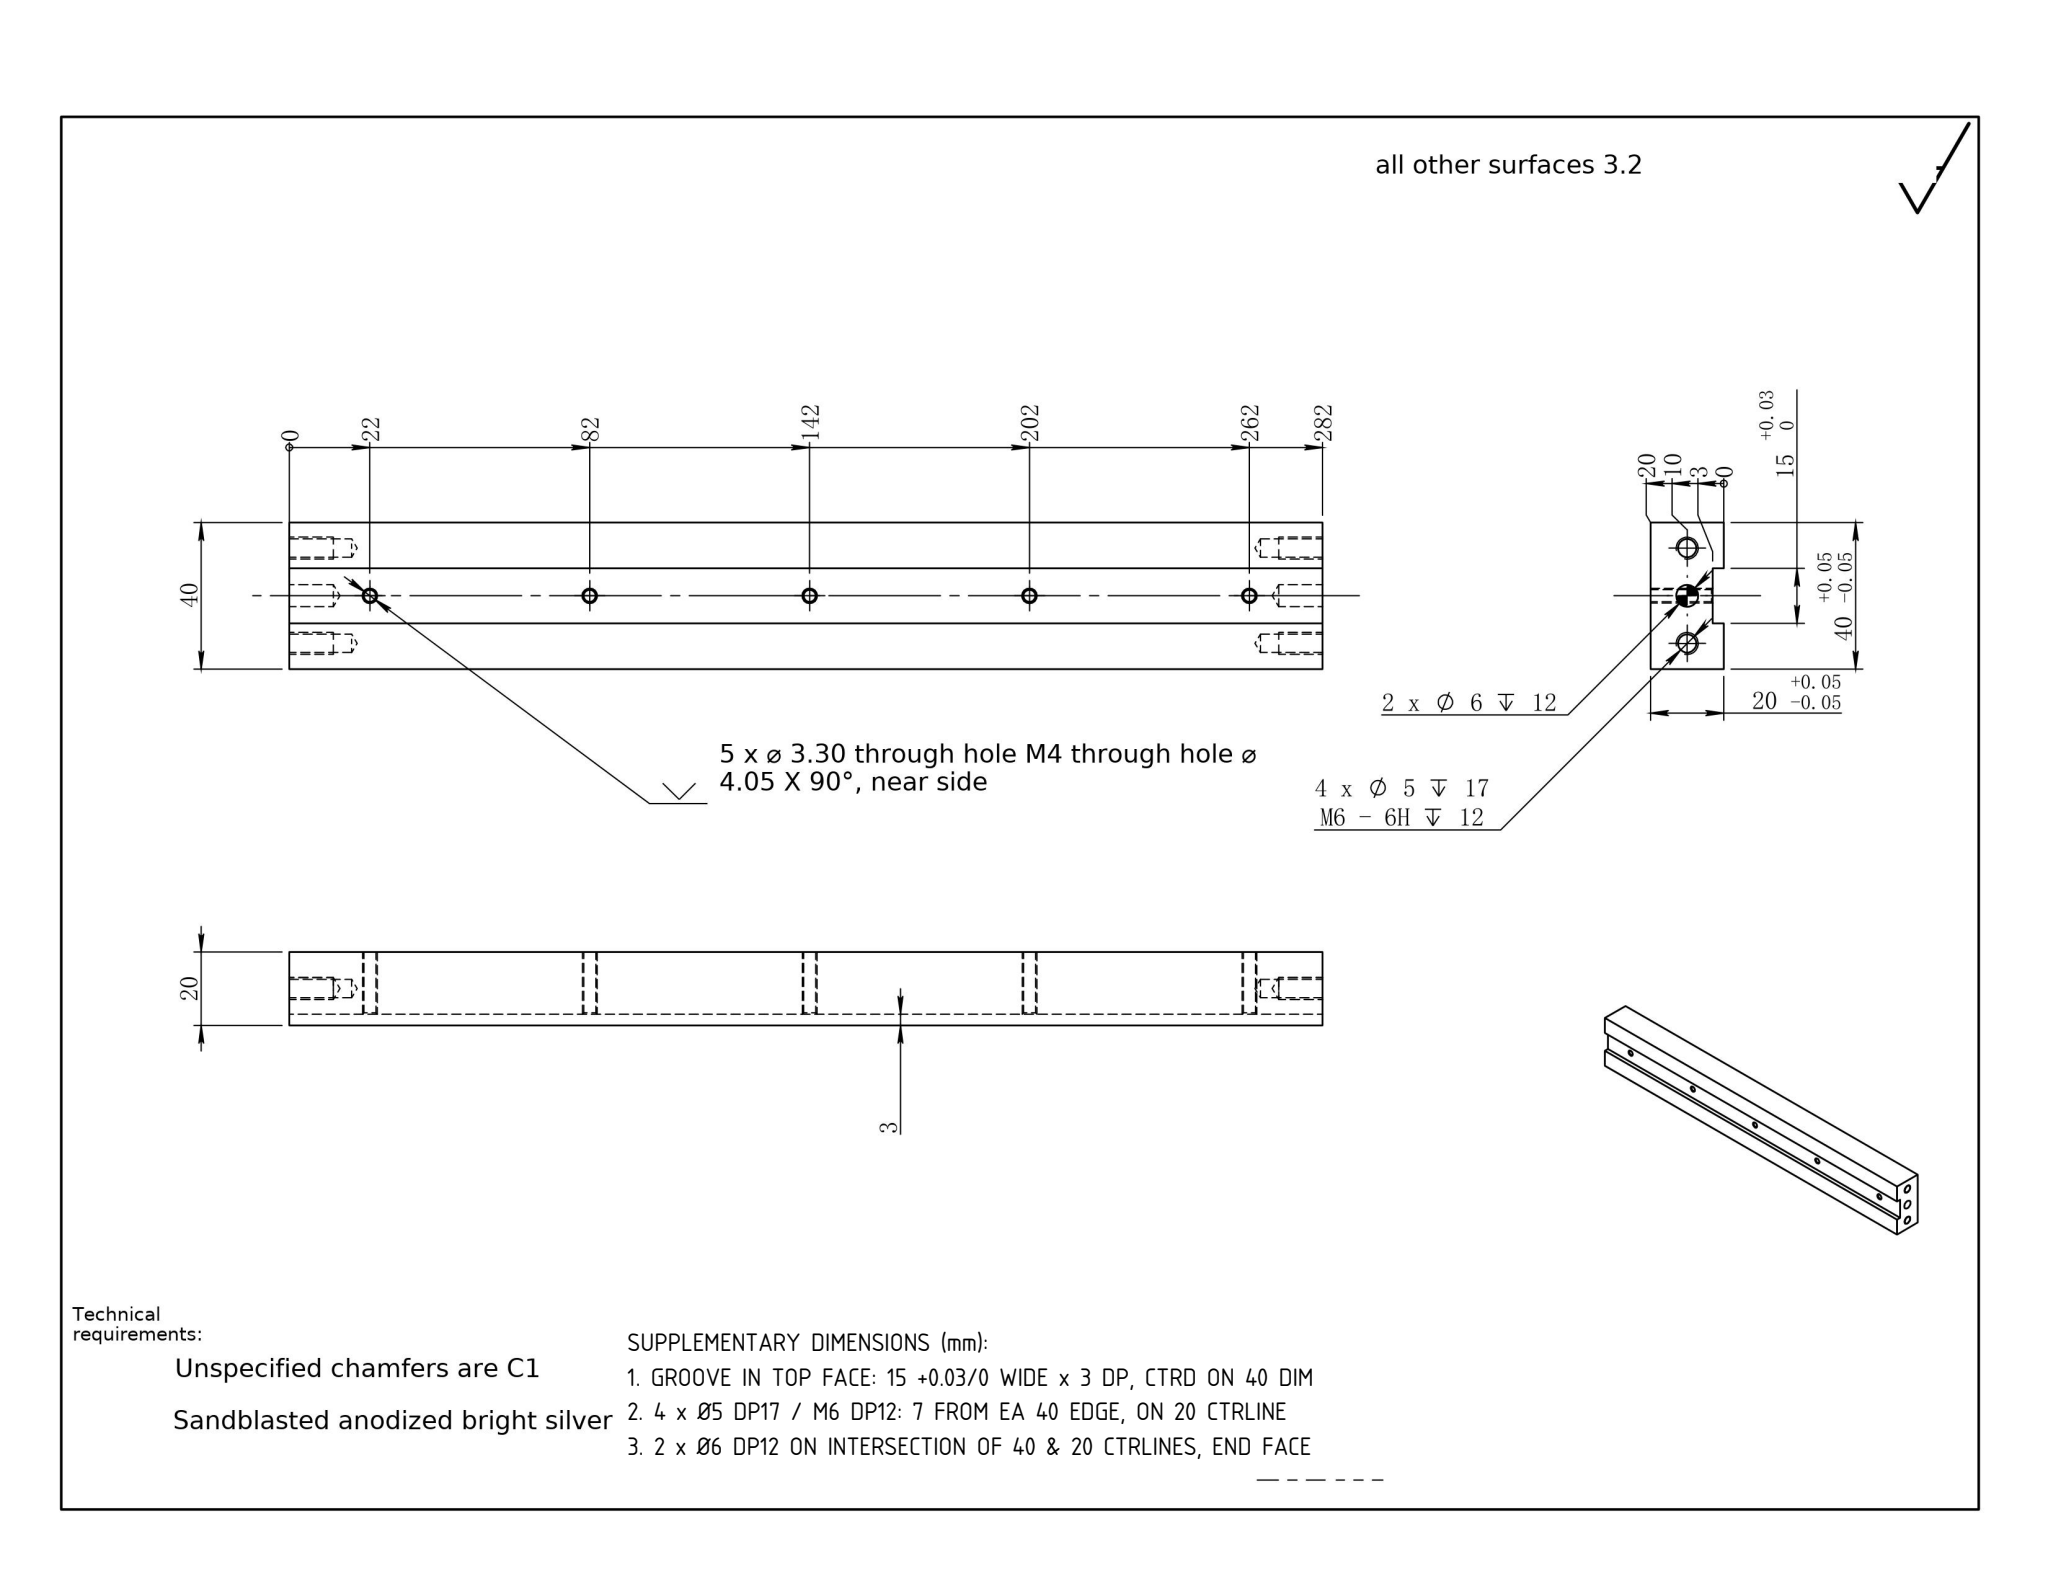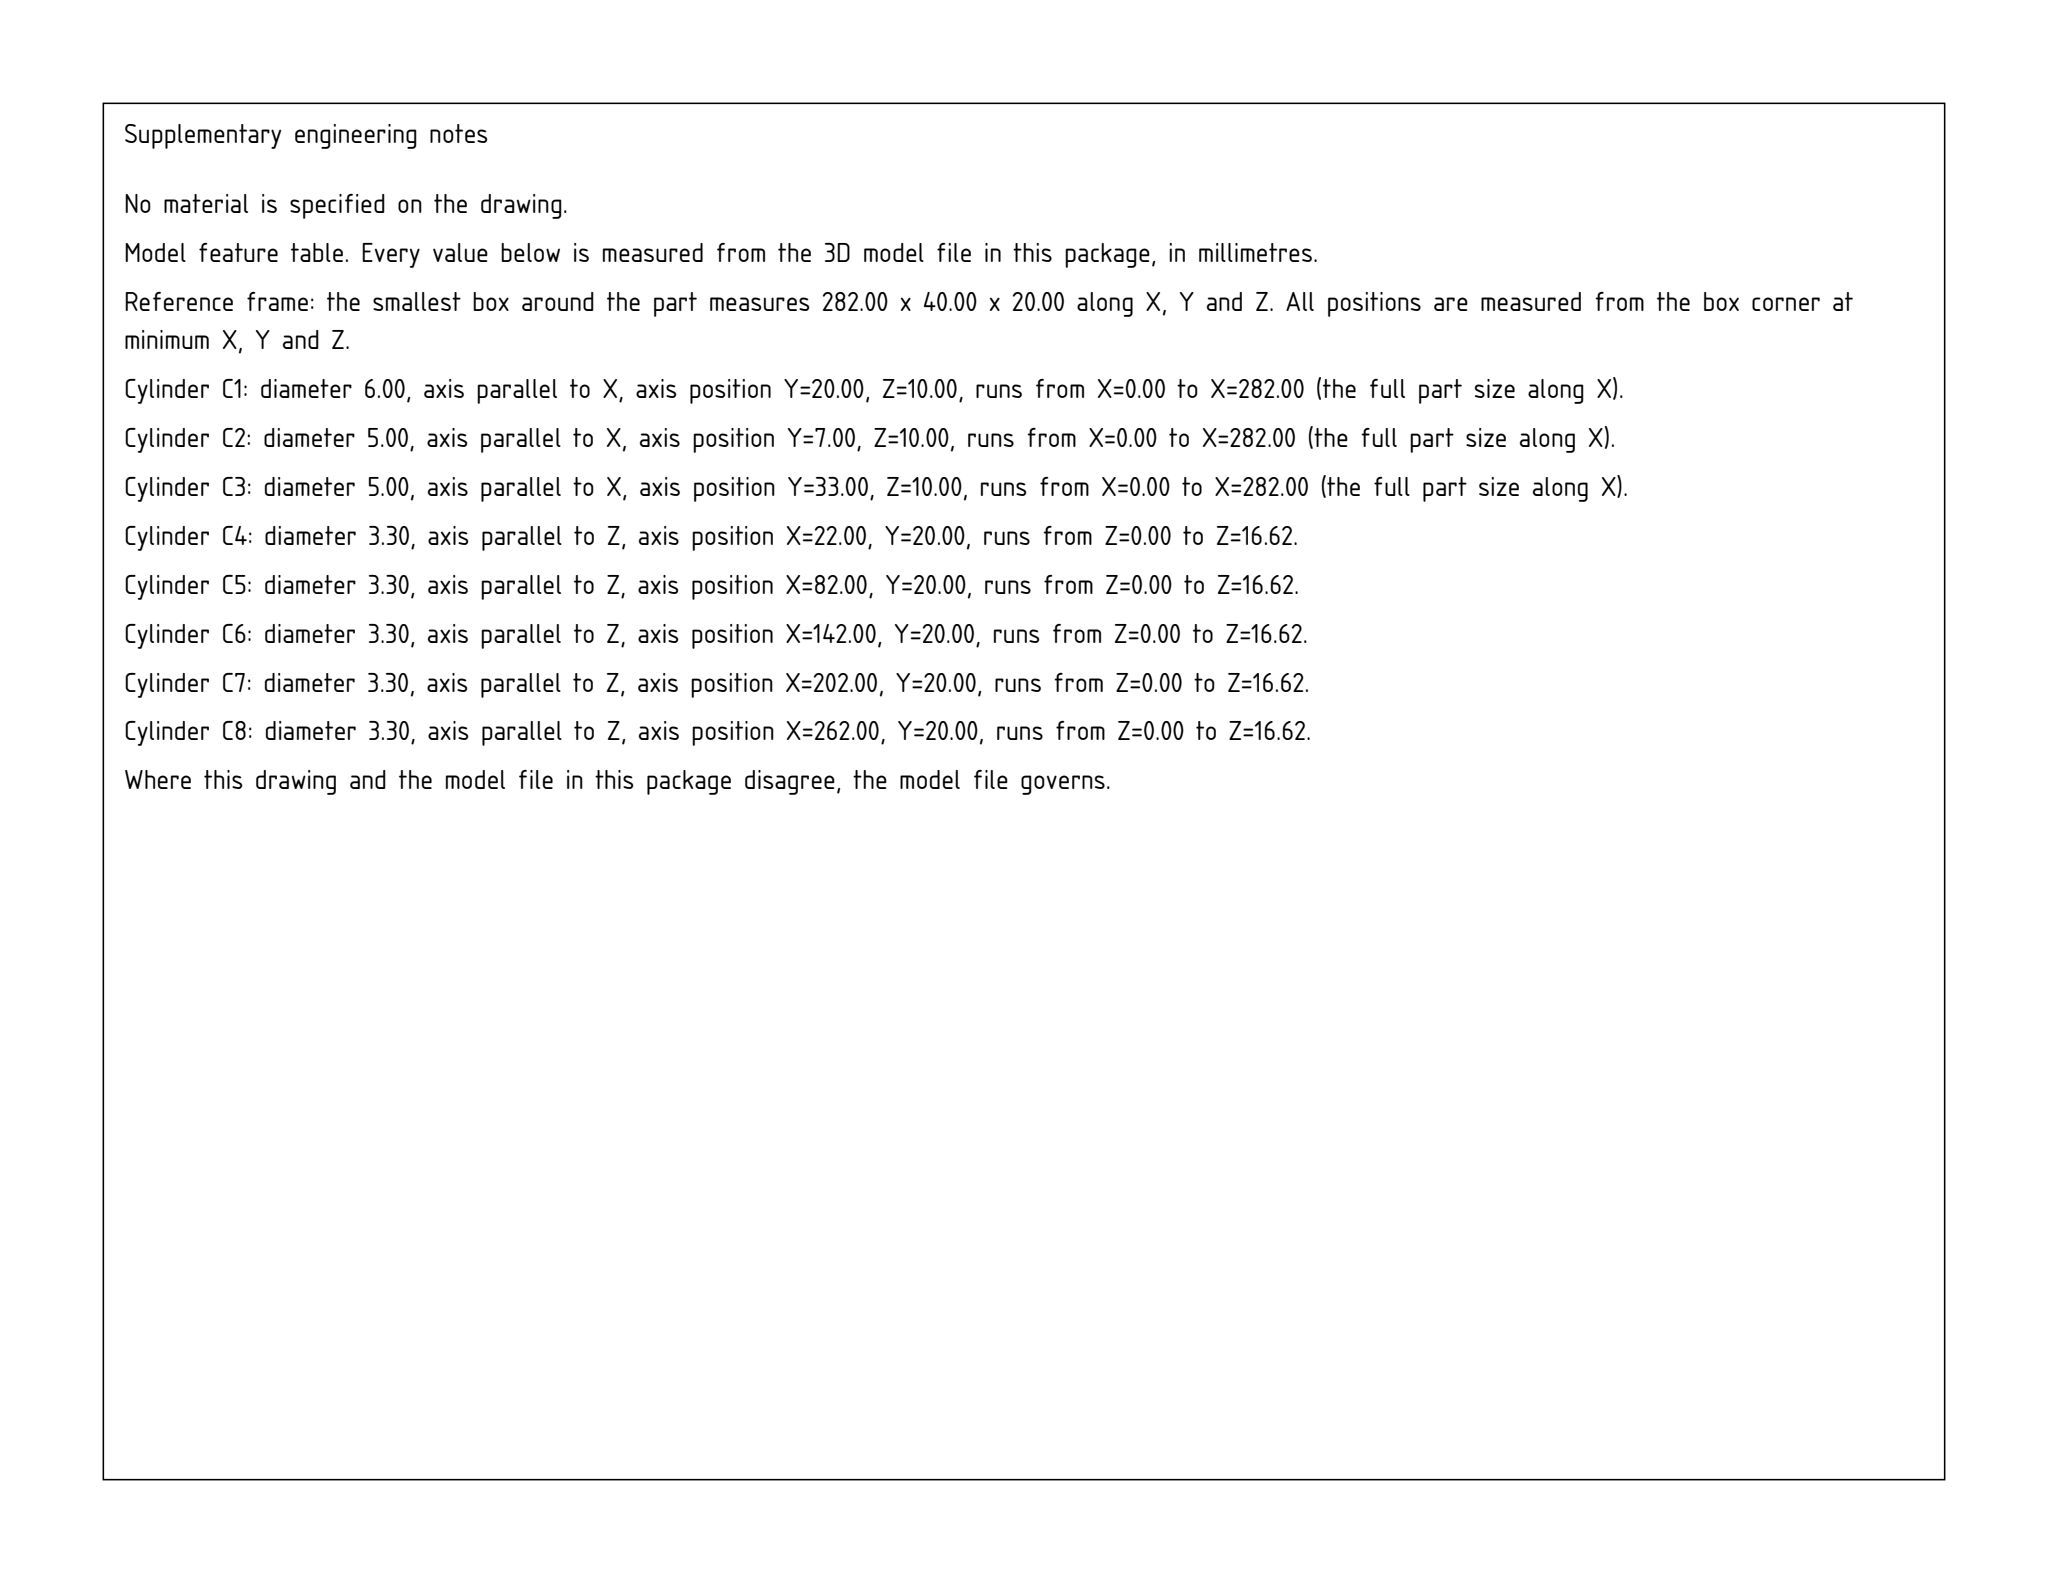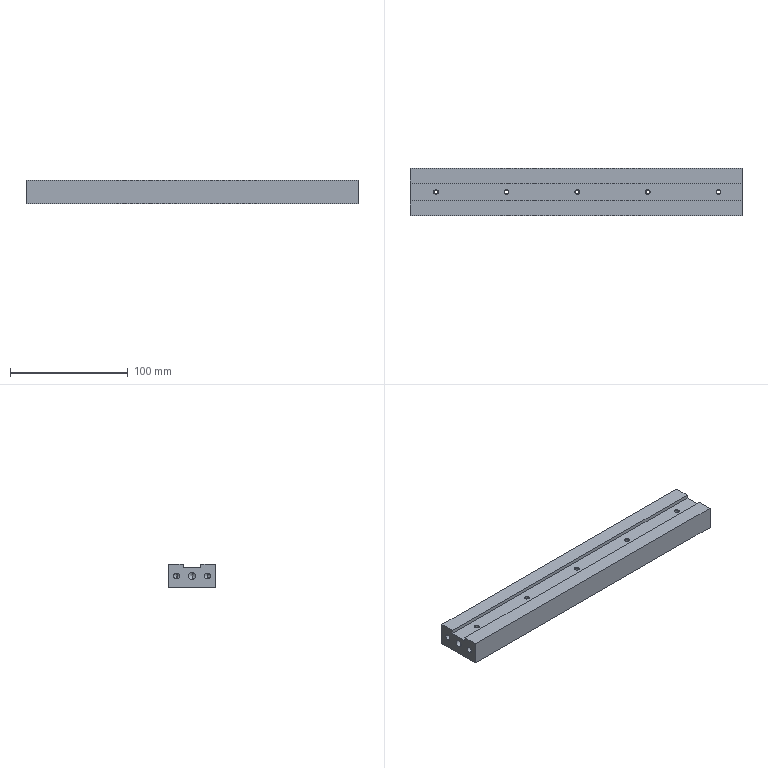Part | SolidWorks | mm | 1 solid | 54 faces | box 282 x 40 x 20 mm | volume 210092 mm3 | cylinder 22 | cone 22 | plane 10 | commonest cylinder face diameters 3.3 x10 5 x8 6 x4
build123d program:
from build123d import *

# Parameters (mm, degrees)
SKETCH1_W                   = 20
SKETCH1_H                   = 40
BOSS_EXTRUDE1_DEPTH         = 141
SKETCH3_W                   = 282
SKETCH3_H                   = 15
CUT_EXTRUDE2_DEPTH          = 3
M4_TAPPED_HOLE1_D           = 3.3
M4_TAPPED_HOLE1_CSINK_D     = 4.05
M4_TAPPED_HOLE1_CSINK_ANGLE = 90
LPATTERN1_COUNT             = 5
LPATTERN1_PITCH             = 60
M6_TAPPED_HOLE1_AT_2_COUNT  = 2
M6_TAPPED_HOLE1_AT_2_PITCH  = 26


with BuildPart() as part:
    # Sketch1 → Boss-Extrude1 (new, symmetric)
    with BuildSketch(Plane(origin=(0, 0, 0), x_dir=(0, 0, -1), z_dir=(1, 0, 0))):
        Rectangle(SKETCH1_W, SKETCH1_H)
    extrude(amount=BOSS_EXTRUDE1_DEPTH, both=True)

    # Sketch3 → Cut-Extrude2 (cut)
    with BuildSketch(Plane(origin=(0, -40, 10), x_dir=(1, 0, 0), z_dir=(0, 0, -1))):
        with Locations((0, -40)):
            Rectangle(SKETCH3_W, SKETCH3_H)
    extrude(amount=CUT_EXTRUDE2_DEPTH, mode=Mode.SUBTRACT)

    # M4 Tapped Hole1 (through all)
    with Locations(Plane.XY.offset(7)):
        with Locations((-119, 0)):
            m4_tapped_hole1 = CounterSinkHole(M4_TAPPED_HOLE1_D / 2, M4_TAPPED_HOLE1_CSINK_D / 2, counter_sink_angle=M4_TAPPED_HOLE1_CSINK_ANGLE)

    # LPattern1: M4 Tapped Hole1 ×5
    with Locations(*[(i * LPATTERN1_PITCH, 0, 0) for i in range(1, LPATTERN1_COUNT)]):
        add(m4_tapped_hole1, mode=Mode.SUBTRACT)

    # Sketch9 → M6 Tapped Hole1 (revolve, cut)
    with BuildSketch(Plane(origin=(141, 13, 0), x_dir=(0, 0, -1), z_dir=(0, 1, 0))):
        Polygon((0, 0), (0, 18.502), (2.5, 17), (2.5, 0), align=None)
    m6_tapped_hole1 = revolve(axis=Axis((147.35, 13, 0), (-1, 0, 0)), mode=Mode.SUBTRACT)

    # M6 Tapped Hole1 at 2: M6 Tapped Hole1 ×2
    with Locations(*[(0, -i * M6_TAPPED_HOLE1_AT_2_PITCH, 0) for i in range(1, M6_TAPPED_HOLE1_AT_2_COUNT)]):
        add(m6_tapped_hole1, mode=Mode.SUBTRACT)

    # Sketch12 → 6.0 _6_ Diameter Hole1 (revolve, cut)
    with BuildSketch(Plane(origin=(141, 0, 0), x_dir=(0, 0, -1), z_dir=(0, 1, 0))):
        Polygon((0, 0), (0, 13.803), (3, 12), (3, 0), align=None)
    f_6_0_6_diameter_hole1 = revolve(axis=Axis((147.35, 0, 0), (-1, 0, 0)), mode=Mode.SUBTRACT)

    # Mirror1: M6 Tapped Hole1, 6.0 _6_ Diameter Hole1 across plane
    add(m6_tapped_hole1.mirror(Plane(origin=(0, 0, 0), x_dir=(0, 0, 1), z_dir=(1, 0, 0))), mode=Mode.SUBTRACT)
    add(f_6_0_6_diameter_hole1.mirror(Plane(origin=(0, 0, 0), x_dir=(0, 0, 1), z_dir=(1, 0, 0))), mode=Mode.SUBTRACT)

    # Mirror1 copy 1 sketch → Mirror1 copy 1 (revolve, cut)
    with BuildSketch(Plane(origin=(-141, -13, 0), x_dir=(0, 0, -1), z_dir=(0, 1, 0))):
        Polygon((0, 0), (0, -18.502), (2.5, -17), (2.5, 0), align=None)
    revolve(axis=Axis((-147.35, -13, 0), (-1, 0, 0)), mode=Mode.SUBTRACT)


solid = part.part